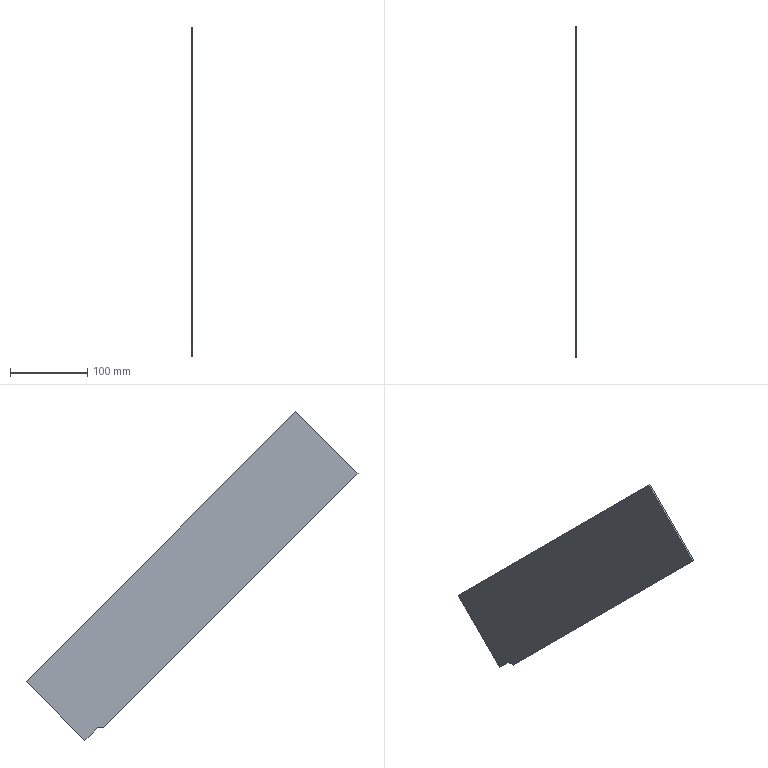Component | SolidWorks | LeftSideGuardPlate-1 | 1 solid | 8 faces | box 2 x 430.63 x 426.39 mm | volume 112548 mm3 | plane 8
build123d program:
from build123d import *

# Parameters (mm, degrees)
SKETCH1_W                              = 495
SKETCH1_H                              = 114
BOSS_EXTRUDE1_DEPTH                    = 2
GUARD_CORNER_CLEARANCE_TOOL_BODY_DEPTH = 3


with BuildPart() as part:
    # Sketch1 → Boss-Extrude1 (new body)
    with BuildSketch(Plane.XY):
        with Locations((180.734, 8.86)):
            Rectangle(SKETCH1_W, SKETCH1_H)
    extrude(amount=BOSS_EXTRUDE1_DEPTH)


with BuildPart() as body_2:
    # Guard Corner Clearance Sketch → Guard Corner Clearance Tool Body (new, symmetric)
    with BuildSketch(Plane.XY):
        Polygon((-30.932, -55), (-43.792, -42.14), (-75, -42.14), (-75, -55), align=None)
    extrude(amount=GUARD_CORNER_CLEARANCE_TOOL_BODY_DEPTH, both=True)


with BuildPart() as part_1:
    add(part.part)

    # Guard 2 and 3 Corner Clearance: cut body 2
    add(body_2.part, mode=Mode.SUBTRACT)


solid = part_1.part

# Placed as in the assembly
solid = solid.moved(Location((-16.175, 84.044, -286.697), (45, -90, 0)))
STEP:
#1=COLOUR_RGB('',0.7922,0.8196,0.9333);
#2=FILL_AREA_STYLE_COLOUR('',#1);
#3=FILL_AREA_STYLE('',(#2));
#4=SURFACE_STYLE_FILL_AREA(#3);
#5=SURFACE_SIDE_STYLE('',(#4));
#6=SURFACE_STYLE_USAGE(.BOTH.,#5);
#7=PRESENTATION_STYLE_ASSIGNMENT((#6));
#8=CARTESIAN_POINT('',(-0.7156,3.994,-14.319));
#9=VERTEX_POINT('',#8);
#10=CARTESIAN_POINT('',(-0.6368,3.994,-14.319));
#11=VERTEX_POINT('',#10);
#12=CARTESIAN_POINT('',(-0.7156,3.994,-14.319));
#13=DIRECTION('',(1.,-0.,0.));
#14=VECTOR('',#13,39.37);
#15=LINE('',#12,#14);
#16=EDGE_CURVE('',#9,#11,#15,.T.);
#17=ORIENTED_EDGE('',*,*,#16,.F.);
#18=CARTESIAN_POINT('',(-0.7156,7.001,-11.313));
#19=VERTEX_POINT('',#18);
#20=CARTESIAN_POINT('',(-0.7156,7.001,-11.313));
#21=DIRECTION('',(-0.,-0.7071,-0.7071));
#22=VECTOR('',#21,39.37);
#23=LINE('',#20,#22);
#24=EDGE_CURVE('',#19,#9,#23,.T.);
#25=ORIENTED_EDGE('',*,*,#24,.F.);
#26=CARTESIAN_POINT('',(-0.6368,7.001,-11.313));
#27=VERTEX_POINT('',#26);
#28=CARTESIAN_POINT('',(-0.7156,7.001,-11.313));
#29=DIRECTION('',(1.,-0.,0.));
#30=VECTOR('',#29,39.37);
#31=LINE('',#28,#30);
#32=EDGE_CURVE('',#19,#27,#31,.T.);
#33=ORIENTED_EDGE('',*,*,#32,.T.);
#34=CARTESIAN_POINT('',(-0.6368,7.001,-11.313));
#35=DIRECTION('',(-0.,-0.7071,-0.7071));
#36=VECTOR('',#35,39.37);
#37=LINE('',#34,#36);
#38=EDGE_CURVE('',#27,#11,#37,.T.);
#39=ORIENTED_EDGE('',*,*,#38,.T.);
#40=EDGE_LOOP('',(#17,#25,#33,#39));
#41=FACE_OUTER_BOUND('',#40,.T.);
#42=CARTESIAN_POINT('',(-0.7156,7.001,-11.313));
#43=DIRECTION('',(-0.,-0.7071,0.7071));
#44=DIRECTION('',(1.,-0.,0.));
#45=AXIS2_PLACEMENT_3D('',#42,#43,#44);
#46=PLANE('',#45);
#47=ADVANCED_FACE('',(#41),#46,.F.);
#48=CARTESIAN_POINT('',(-0.6368,3.021,-13.68));
#49=VERTEX_POINT('',#48);
#50=CARTESIAN_POINT('',(-0.7156,3.021,-13.68));
#51=VERTEX_POINT('',#50);
#52=CARTESIAN_POINT('',(-0.7156,3.021,-13.68));
#53=DIRECTION('',(-1.,0.,-0.));
#54=VECTOR('',#53,39.37);
#55=LINE('',#52,#54);
#56=EDGE_CURVE('',#49,#51,#55,.T.);
#57=ORIENTED_EDGE('',*,*,#56,.F.);
#58=CARTESIAN_POINT('',(-0.6368,-9.953,-0.7059));
#59=VERTEX_POINT('',#58);
#60=CARTESIAN_POINT('',(-0.6368,3.827,-14.486));
#61=DIRECTION('',(-0.,-0.7071,0.7071));
#62=VECTOR('',#61,39.37);
#63=LINE('',#60,#62);
#64=EDGE_CURVE('',#49,#59,#63,.T.);
#65=ORIENTED_EDGE('',*,*,#64,.T.);
#66=CARTESIAN_POINT('',(-0.7156,-9.953,-0.7059));
#67=VERTEX_POINT('',#66);
#68=CARTESIAN_POINT('',(-0.7156,-9.953,-0.7059));
#69=DIRECTION('',(1.,-0.,0.));
#70=VECTOR('',#69,39.37);
#71=LINE('',#68,#70);
#72=EDGE_CURVE('',#67,#59,#71,.T.);
#73=ORIENTED_EDGE('',*,*,#72,.F.);
#74=CARTESIAN_POINT('',(-0.7156,3.827,-14.486));
#75=DIRECTION('',(-0.,-0.7071,0.7071));
#76=VECTOR('',#75,39.37);
#77=LINE('',#74,#76);
#78=EDGE_CURVE('',#51,#67,#77,.T.);
#79=ORIENTED_EDGE('',*,*,#78,.F.);
#80=EDGE_LOOP('',(#57,#65,#73,#79));
#81=FACE_OUTER_BOUND('',#80,.T.);
#82=CARTESIAN_POINT('',(-0.7156,3.827,-14.486));
#83=DIRECTION('',(0.,0.7071,0.7071));
#84=DIRECTION('',(-1.,0.,-0.));
#85=AXIS2_PLACEMENT_3D('',#82,#83,#84);
#86=PLANE('',#85);
#87=ADVANCED_FACE('',(#81),#86,.F.);
#88=CARTESIAN_POINT('',(-0.7156,3.355,-13.68));
#89=VERTEX_POINT('',#88);
#90=CARTESIAN_POINT('',(-0.7156,2.136,-12.46));
#91=DIRECTION('',(-0.,-0.7071,0.7071));
#92=VECTOR('',#91,39.37);
#93=LINE('',#90,#92);
#94=EDGE_CURVE('',#9,#89,#93,.T.);
#95=ORIENTED_EDGE('',*,*,#94,.T.);
#96=CARTESIAN_POINT('',(-0.7156,3.309,-13.68));
#97=DIRECTION('',(-0.,-1.,-0.));
#98=VECTOR('',#97,39.37);
#99=LINE('',#96,#98);
#100=EDGE_CURVE('',#89,#51,#99,.T.);
#101=ORIENTED_EDGE('',*,*,#100,.T.);
#102=ORIENTED_EDGE('',*,*,#78,.T.);
#103=CARTESIAN_POINT('',(-0.7156,-6.779,2.468));
#104=VERTEX_POINT('',#103);
#105=CARTESIAN_POINT('',(-0.7156,-6.779,2.468));
#106=DIRECTION('',(0.,0.7071,0.7071));
#107=VECTOR('',#106,39.37);
#108=LINE('',#105,#107);
#109=EDGE_CURVE('',#67,#104,#108,.T.);
#110=ORIENTED_EDGE('',*,*,#109,.T.);
#111=CARTESIAN_POINT('',(-0.7156,7.001,-11.313));
#112=DIRECTION('',(0.,0.7071,-0.7071));
#113=VECTOR('',#112,39.37);
#114=LINE('',#111,#113);
#115=EDGE_CURVE('',#104,#19,#114,.T.);
#116=ORIENTED_EDGE('',*,*,#115,.T.);
#117=ORIENTED_EDGE('',*,*,#24,.T.);
#118=EDGE_LOOP('',(#95,#101,#102,#110,#116,#117));
#119=FACE_OUTER_BOUND('',#118,.T.);
#120=CARTESIAN_POINT('',(-0.7156,3.309,-11.287));
#121=DIRECTION('',(-1.,0.,-0.));
#122=DIRECTION('',(-0.,-0.7071,0.7071));
#123=AXIS2_PLACEMENT_3D('',#120,#121,#122);
#124=PLANE('',#123);
#125=ADVANCED_FACE('',(#119),#124,.T.);
#126=CARTESIAN_POINT('',(-0.6368,3.355,-13.68));
#127=VERTEX_POINT('',#126);
#128=CARTESIAN_POINT('',(-0.6368,3.309,-13.68));
#129=DIRECTION('',(-0.,-1.,-0.));
#130=VECTOR('',#129,39.37);
#131=LINE('',#128,#130);
#132=EDGE_CURVE('',#127,#49,#131,.T.);
#133=ORIENTED_EDGE('',*,*,#132,.F.);
#134=CARTESIAN_POINT('',(-0.6368,2.136,-12.46));
#135=DIRECTION('',(-0.,-0.7071,0.7071));
#136=VECTOR('',#135,39.37);
#137=LINE('',#134,#136);
#138=EDGE_CURVE('',#11,#127,#137,.T.);
#139=ORIENTED_EDGE('',*,*,#138,.F.);
#140=ORIENTED_EDGE('',*,*,#38,.F.);
#141=CARTESIAN_POINT('',(-0.6368,-6.779,2.468));
#142=VERTEX_POINT('',#141);
#143=CARTESIAN_POINT('',(-0.6368,7.001,-11.313));
#144=DIRECTION('',(0.,0.7071,-0.7071));
#145=VECTOR('',#144,39.37);
#146=LINE('',#143,#145);
#147=EDGE_CURVE('',#142,#27,#146,.T.);
#148=ORIENTED_EDGE('',*,*,#147,.F.);
#149=CARTESIAN_POINT('',(-0.6368,-6.779,2.468));
#150=DIRECTION('',(0.,0.7071,0.7071));
#151=VECTOR('',#150,39.37);
#152=LINE('',#149,#151);
#153=EDGE_CURVE('',#59,#142,#152,.T.);
#154=ORIENTED_EDGE('',*,*,#153,.F.);
#155=ORIENTED_EDGE('',*,*,#64,.F.);
#156=EDGE_LOOP('',(#133,#139,#140,#148,#154,#155));
#157=FACE_OUTER_BOUND('',#156,.T.);
#158=CARTESIAN_POINT('',(-0.6368,3.309,-11.287));
#159=DIRECTION('',(-1.,0.,-0.));
#160=DIRECTION('',(-0.,-0.7071,0.7071));
#161=AXIS2_PLACEMENT_3D('',#158,#159,#160);
#162=PLANE('',#161);
#163=ADVANCED_FACE('',(#157),#162,.F.);
#164=ORIENTED_EDGE('',*,*,#153,.T.);
#165=CARTESIAN_POINT('',(-0.7156,-6.779,2.468));
#166=DIRECTION('',(1.,-0.,0.));
#167=VECTOR('',#166,39.37);
#168=LINE('',#165,#167);
#169=EDGE_CURVE('',#104,#142,#168,.T.);
#170=ORIENTED_EDGE('',*,*,#169,.F.);
#171=ORIENTED_EDGE('',*,*,#109,.F.);
#172=ORIENTED_EDGE('',*,*,#72,.T.);
#173=EDGE_LOOP('',(#164,#170,#171,#172));
#174=FACE_OUTER_BOUND('',#173,.T.);
#175=CARTESIAN_POINT('',(-0.7156,-6.779,2.468));
#176=DIRECTION('',(0.,0.7071,-0.7071));
#177=DIRECTION('',(-0.,-0.7071,-0.7071));
#178=AXIS2_PLACEMENT_3D('',#175,#176,#177);
#179=PLANE('',#178);
#180=ADVANCED_FACE('',(#174),#179,.F.);
#181=ORIENTED_EDGE('',*,*,#147,.T.);
#182=ORIENTED_EDGE('',*,*,#32,.F.);
#183=ORIENTED_EDGE('',*,*,#115,.F.);
#184=ORIENTED_EDGE('',*,*,#169,.T.);
#185=EDGE_LOOP('',(#181,#182,#183,#184));
#186=FACE_OUTER_BOUND('',#185,.T.);
#187=CARTESIAN_POINT('',(-0.7156,7.001,-11.313));
#188=DIRECTION('',(-0.,-0.7071,-0.7071));
#189=DIRECTION('',(1.,-0.,0.));
#190=AXIS2_PLACEMENT_3D('',#187,#188,#189);
#191=PLANE('',#190);
#192=ADVANCED_FACE('',(#186),#191,.F.);
#193=CARTESIAN_POINT('',(-0.7549,3.355,-13.68));
#194=DIRECTION('',(1.,-0.,0.));
#195=VECTOR('',#194,39.37);
#196=LINE('',#193,#195);
#197=EDGE_CURVE('',#89,#127,#196,.T.);
#198=ORIENTED_EDGE('',*,*,#197,.T.);
#199=ORIENTED_EDGE('',*,*,#132,.T.);
#200=ORIENTED_EDGE('',*,*,#56,.T.);
#201=ORIENTED_EDGE('',*,*,#100,.F.);
#202=EDGE_LOOP('',(#198,#199,#200,#201));
#203=FACE_OUTER_BOUND('',#202,.T.);
#204=CARTESIAN_POINT('',(-0.7549,2.639,-13.68));
#205=DIRECTION('',(0.,0.,-1.));
#206=DIRECTION('',(-0.,-1.,-0.));
#207=AXIS2_PLACEMENT_3D('',#204,#205,#206);
#208=PLANE('',#207);
#209=ADVANCED_FACE('',(#203),#208,.T.);
#210=ORIENTED_EDGE('',*,*,#16,.T.);
#211=ORIENTED_EDGE('',*,*,#138,.T.);
#212=ORIENTED_EDGE('',*,*,#197,.F.);
#213=ORIENTED_EDGE('',*,*,#94,.F.);
#214=EDGE_LOOP('',(#210,#211,#212,#213));
#215=FACE_OUTER_BOUND('',#214,.T.);
#216=CARTESIAN_POINT('',(-0.7549,3.355,-13.68));
#217=DIRECTION('',(-0.,-0.7071,-0.7071));
#218=DIRECTION('',(1.,-0.,0.));
#219=AXIS2_PLACEMENT_3D('',#216,#217,#218);
#220=PLANE('',#219);
#221=ADVANCED_FACE('',(#215),#220,.T.);
#222=CLOSED_SHELL('',(#47,#87,#125,#163,#180,#192,#209,#221));
#223=MANIFOLD_SOLID_BREP('',#222);
#224=STYLED_ITEM('',(#7),#223);
#225=(LENGTH_UNIT()NAMED_UNIT(*)SI_UNIT($,.METRE.));
#226=LENGTH_MEASURE_WITH_UNIT(LENGTH_MEASURE(0.0254),#225);
#227=DIMENSIONAL_EXPONENTS(1.,0.,0.,0.,0.,0.,0.);
#228=(CONVERSION_BASED_UNIT('',#226)LENGTH_UNIT()NAMED_UNIT(#227));
#229=UNCERTAINTY_MEASURE_WITH_UNIT(LENGTH_MEASURE(0.00001),#228,'','');
#230=(NAMED_UNIT(*)PLANE_ANGLE_UNIT()SI_UNIT($,.RADIAN.));
#231=(NAMED_UNIT(*)SI_UNIT($,.STERADIAN.)SOLID_ANGLE_UNIT());
#232=(GEOMETRIC_REPRESENTATION_CONTEXT(3)GLOBAL_UNCERTAINTY_ASSIGNED_CONTEXT((#229))GLOBAL_UNIT_ASSIGNED_CONTEXT((#228,#230,#231))REPRESENTATION_CONTEXT('',''));
#233=MECHANICAL_DESIGN_GEOMETRIC_PRESENTATION_REPRESENTATION('',(#224),#232);
#234=CARTESIAN_POINT('',(0.,0.,0.));
#235=DIRECTION('',(0.,0.,1.));
#236=DIRECTION('',(1.,0.,0.));
#237=AXIS2_PLACEMENT_3D('',#234,#235,#236);
#238=(LENGTH_UNIT()NAMED_UNIT(*)SI_UNIT($,.METRE.));
#239=LENGTH_MEASURE_WITH_UNIT(LENGTH_MEASURE(0.0254),#238);
#240=DIMENSIONAL_EXPONENTS(1.,0.,0.,0.,0.,0.,0.);
#241=(CONVERSION_BASED_UNIT('',#239)LENGTH_UNIT()NAMED_UNIT(#240));
#242=UNCERTAINTY_MEASURE_WITH_UNIT(LENGTH_MEASURE(0.00001),#241,'','');
#243=(NAMED_UNIT(*)PLANE_ANGLE_UNIT()SI_UNIT($,.RADIAN.));
#244=(NAMED_UNIT(*)SI_UNIT($,.STERADIAN.)SOLID_ANGLE_UNIT());
#245=(GEOMETRIC_REPRESENTATION_CONTEXT(3)GLOBAL_UNCERTAINTY_ASSIGNED_CONTEXT((#242))GLOBAL_UNIT_ASSIGNED_CONTEXT((#241,#243,#244))REPRESENTATION_CONTEXT('',''));
#246=ADVANCED_BREP_SHAPE_REPRESENTATION('',(#223,#237),#245);
#247=PRESENTATION_LAYER_ASSIGNMENT('','',(#224));